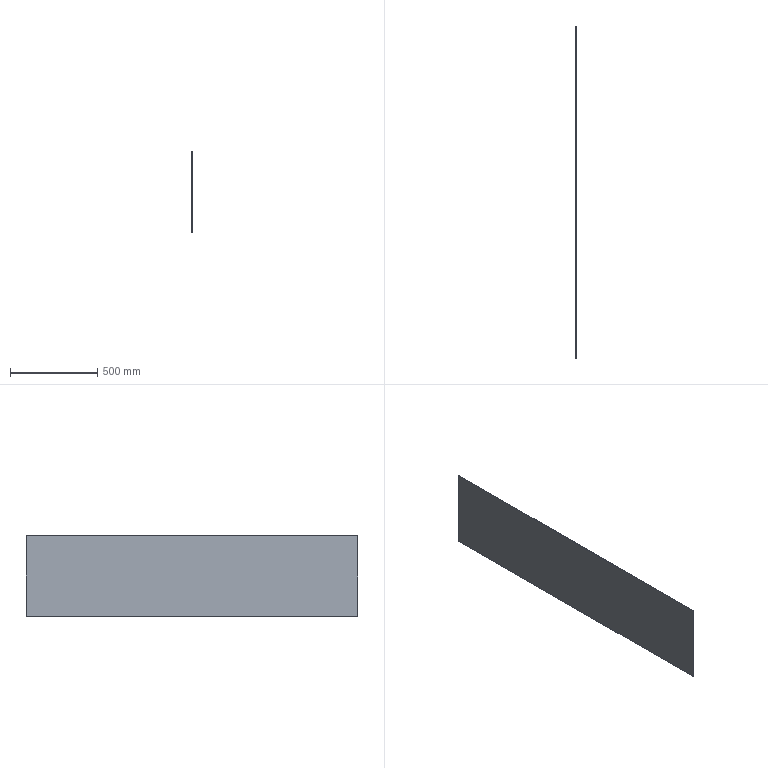Component | SolidWorks | SideBottomPlate-1 | 1 solid | 6 faces | box 2 x 1900 x 460 mm | volume 1748000 mm3 | plane 6 | material Plain Carbon Steel
STEP:
#1=CARTESIAN_POINT('',(-18.861,73.955,-5.218));
#2=VERTEX_POINT('',#1);
#3=CARTESIAN_POINT('',(-18.861,-0.848,-5.218));
#4=VERTEX_POINT('',#3);
#5=CARTESIAN_POINT('',(-18.861,73.955,-5.218));
#6=DIRECTION('',(-0.,-1.,0.));
#7=VECTOR('',#6,39.37);
#8=LINE('',#5,#7);
#9=EDGE_CURVE('',#2,#4,#8,.T.);
#10=ORIENTED_EDGE('',*,*,#9,.F.);
#11=CARTESIAN_POINT('',(-18.782,73.955,-5.218));
#12=VERTEX_POINT('',#11);
#13=CARTESIAN_POINT('',(-18.782,73.955,-5.218));
#14=DIRECTION('',(-1.,0.,-0.));
#15=VECTOR('',#14,39.37);
#16=LINE('',#13,#15);
#17=EDGE_CURVE('',#12,#2,#16,.T.);
#18=ORIENTED_EDGE('',*,*,#17,.F.);
#19=CARTESIAN_POINT('',(-18.782,-0.848,-5.218));
#20=VERTEX_POINT('',#19);
#21=CARTESIAN_POINT('',(-18.782,73.955,-5.218));
#22=DIRECTION('',(-0.,-1.,0.));
#23=VECTOR('',#22,39.37);
#24=LINE('',#21,#23);
#25=EDGE_CURVE('',#12,#20,#24,.T.);
#26=ORIENTED_EDGE('',*,*,#25,.T.);
#27=CARTESIAN_POINT('',(-18.782,-0.848,-5.218));
#28=DIRECTION('',(-1.,0.,-0.));
#29=VECTOR('',#28,39.37);
#30=LINE('',#27,#29);
#31=EDGE_CURVE('',#20,#4,#30,.T.);
#32=ORIENTED_EDGE('',*,*,#31,.T.);
#33=EDGE_LOOP('',(#10,#18,#26,#32));
#34=FACE_OUTER_BOUND('',#33,.T.);
#35=CARTESIAN_POINT('',(-18.782,73.955,-5.218));
#36=DIRECTION('',(0.,-0.,-1.));
#37=DIRECTION('',(-0.,-1.,0.));
#38=AXIS2_PLACEMENT_3D('',#35,#36,#37);
#39=PLANE('',#38);
#40=ADVANCED_FACE('',(#34),#39,.T.);
#41=CARTESIAN_POINT('',(-18.861,73.955,12.893));
#42=VERTEX_POINT('',#41);
#43=CARTESIAN_POINT('',(-18.861,73.955,-5.218));
#44=DIRECTION('',(0.,-0.,-1.));
#45=VECTOR('',#44,39.37);
#46=LINE('',#43,#45);
#47=EDGE_CURVE('',#42,#2,#46,.T.);
#48=ORIENTED_EDGE('',*,*,#47,.F.);
#49=CARTESIAN_POINT('',(-18.782,73.955,12.893));
#50=VERTEX_POINT('',#49);
#51=CARTESIAN_POINT('',(-18.782,73.955,12.893));
#52=DIRECTION('',(-1.,0.,-0.));
#53=VECTOR('',#52,39.37);
#54=LINE('',#51,#53);
#55=EDGE_CURVE('',#50,#42,#54,.T.);
#56=ORIENTED_EDGE('',*,*,#55,.F.);
#57=CARTESIAN_POINT('',(-18.782,73.955,-5.218));
#58=DIRECTION('',(0.,-0.,-1.));
#59=VECTOR('',#58,39.37);
#60=LINE('',#57,#59);
#61=EDGE_CURVE('',#50,#12,#60,.T.);
#62=ORIENTED_EDGE('',*,*,#61,.T.);
#63=ORIENTED_EDGE('',*,*,#17,.T.);
#64=EDGE_LOOP('',(#48,#56,#62,#63));
#65=FACE_OUTER_BOUND('',#64,.T.);
#66=CARTESIAN_POINT('',(-18.782,73.955,-5.218));
#67=DIRECTION('',(0.,1.,-0.));
#68=DIRECTION('',(-1.,0.,-0.));
#69=AXIS2_PLACEMENT_3D('',#66,#67,#68);
#70=PLANE('',#69);
#71=ADVANCED_FACE('',(#65),#70,.T.);
#72=CARTESIAN_POINT('',(-18.861,-0.848,12.893));
#73=VERTEX_POINT('',#72);
#74=CARTESIAN_POINT('',(-18.861,73.955,12.893));
#75=DIRECTION('',(0.,1.,-0.));
#76=VECTOR('',#75,39.37);
#77=LINE('',#74,#76);
#78=EDGE_CURVE('',#73,#42,#77,.T.);
#79=ORIENTED_EDGE('',*,*,#78,.F.);
#80=CARTESIAN_POINT('',(-18.782,-0.848,12.893));
#81=VERTEX_POINT('',#80);
#82=CARTESIAN_POINT('',(-18.782,-0.848,12.893));
#83=DIRECTION('',(-1.,0.,-0.));
#84=VECTOR('',#83,39.37);
#85=LINE('',#82,#84);
#86=EDGE_CURVE('',#81,#73,#85,.T.);
#87=ORIENTED_EDGE('',*,*,#86,.F.);
#88=CARTESIAN_POINT('',(-18.782,73.955,12.893));
#89=DIRECTION('',(0.,1.,-0.));
#90=VECTOR('',#89,39.37);
#91=LINE('',#88,#90);
#92=EDGE_CURVE('',#81,#50,#91,.T.);
#93=ORIENTED_EDGE('',*,*,#92,.T.);
#94=ORIENTED_EDGE('',*,*,#55,.T.);
#95=EDGE_LOOP('',(#79,#87,#93,#94));
#96=FACE_OUTER_BOUND('',#95,.T.);
#97=CARTESIAN_POINT('',(-18.782,73.955,12.893));
#98=DIRECTION('',(-0.,0.,1.));
#99=DIRECTION('',(0.,1.,-0.));
#100=AXIS2_PLACEMENT_3D('',#97,#98,#99);
#101=PLANE('',#100);
#102=ADVANCED_FACE('',(#96),#101,.T.);
#103=CARTESIAN_POINT('',(-18.861,-0.848,-5.218));
#104=DIRECTION('',(-0.,0.,1.));
#105=VECTOR('',#104,39.37);
#106=LINE('',#103,#105);
#107=EDGE_CURVE('',#4,#73,#106,.T.);
#108=ORIENTED_EDGE('',*,*,#107,.F.);
#109=ORIENTED_EDGE('',*,*,#31,.F.);
#110=CARTESIAN_POINT('',(-18.782,-0.848,-5.218));
#111=DIRECTION('',(-0.,0.,1.));
#112=VECTOR('',#111,39.37);
#113=LINE('',#110,#112);
#114=EDGE_CURVE('',#20,#81,#113,.T.);
#115=ORIENTED_EDGE('',*,*,#114,.T.);
#116=ORIENTED_EDGE('',*,*,#86,.T.);
#117=EDGE_LOOP('',(#108,#109,#115,#116));
#118=FACE_OUTER_BOUND('',#117,.T.);
#119=CARTESIAN_POINT('',(-18.782,-0.848,-5.218));
#120=DIRECTION('',(-0.,-1.,0.));
#121=DIRECTION('',(1.,-0.,0.));
#122=AXIS2_PLACEMENT_3D('',#119,#120,#121);
#123=PLANE('',#122);
#124=ADVANCED_FACE('',(#118),#123,.T.);
#125=ORIENTED_EDGE('',*,*,#25,.F.);
#126=ORIENTED_EDGE('',*,*,#61,.F.);
#127=ORIENTED_EDGE('',*,*,#92,.F.);
#128=ORIENTED_EDGE('',*,*,#114,.F.);
#129=EDGE_LOOP('',(#125,#126,#127,#128));
#130=FACE_OUTER_BOUND('',#129,.T.);
#131=CARTESIAN_POINT('',(-18.782,71.776,-1.6));
#132=DIRECTION('',(-1.,0.,-0.));
#133=DIRECTION('',(-0.,0.,1.));
#134=AXIS2_PLACEMENT_3D('',#131,#132,#133);
#135=PLANE('',#134);
#136=ADVANCED_FACE('',(#130),#135,.F.);
#137=ORIENTED_EDGE('',*,*,#9,.T.);
#138=ORIENTED_EDGE('',*,*,#107,.T.);
#139=ORIENTED_EDGE('',*,*,#78,.T.);
#140=ORIENTED_EDGE('',*,*,#47,.T.);
#141=EDGE_LOOP('',(#137,#138,#139,#140));
#142=FACE_OUTER_BOUND('',#141,.T.);
#143=CARTESIAN_POINT('',(-18.861,71.776,-1.6));
#144=DIRECTION('',(-1.,0.,-0.));
#145=DIRECTION('',(-0.,0.,1.));
#146=AXIS2_PLACEMENT_3D('',#143,#144,#145);
#147=PLANE('',#146);
#148=ADVANCED_FACE('',(#142),#147,.T.);
#149=CLOSED_SHELL('',(#40,#71,#102,#124,#136,#148));
#150=MANIFOLD_SOLID_BREP('',#149);
#151=CARTESIAN_POINT('',(0.,0.,0.));
#152=DIRECTION('',(0.,0.,1.));
#153=DIRECTION('',(1.,0.,0.));
#154=AXIS2_PLACEMENT_3D('',#151,#152,#153);
#155=(LENGTH_UNIT()NAMED_UNIT(*)SI_UNIT($,.METRE.));
#156=LENGTH_MEASURE_WITH_UNIT(LENGTH_MEASURE(0.0254),#155);
#157=DIMENSIONAL_EXPONENTS(1.,0.,0.,0.,0.,0.,0.);
#158=(CONVERSION_BASED_UNIT('',#156)LENGTH_UNIT()NAMED_UNIT(#157));
#159=UNCERTAINTY_MEASURE_WITH_UNIT(LENGTH_MEASURE(0.00001),#158,'','');
#160=(NAMED_UNIT(*)PLANE_ANGLE_UNIT()SI_UNIT($,.RADIAN.));
#161=(NAMED_UNIT(*)SI_UNIT($,.STERADIAN.)SOLID_ANGLE_UNIT());
#162=(GEOMETRIC_REPRESENTATION_CONTEXT(3)GLOBAL_UNCERTAINTY_ASSIGNED_CONTEXT((#159))GLOBAL_UNIT_ASSIGNED_CONTEXT((#158,#160,#161))REPRESENTATION_CONTEXT('',''));
#163=ADVANCED_BREP_SHAPE_REPRESENTATION('',(#150,#154),#162);
#164=COLOUR_RGB('',0.7922,0.8196,0.9333);
#165=FILL_AREA_STYLE_COLOUR('',#164);
#166=FILL_AREA_STYLE('',(#165));
#167=SURFACE_STYLE_FILL_AREA(#166);
#168=SURFACE_SIDE_STYLE('',(#167));
#169=SURFACE_STYLE_USAGE(.BOTH.,#168);
#170=PRESENTATION_STYLE_ASSIGNMENT((#169));
#171=STYLED_ITEM('',(#170),#150);
#172=PRESENTATION_LAYER_ASSIGNMENT('','',(#171));
#173=(LENGTH_UNIT()NAMED_UNIT(*)SI_UNIT($,.METRE.));
#174=LENGTH_MEASURE_WITH_UNIT(LENGTH_MEASURE(0.0254),#173);
#175=DIMENSIONAL_EXPONENTS(1.,0.,0.,0.,0.,0.,0.);
#176=(CONVERSION_BASED_UNIT('',#174)LENGTH_UNIT()NAMED_UNIT(#175));
#177=UNCERTAINTY_MEASURE_WITH_UNIT(LENGTH_MEASURE(0.00001),#176,'','');
#178=(NAMED_UNIT(*)PLANE_ANGLE_UNIT()SI_UNIT($,.RADIAN.));
#179=(NAMED_UNIT(*)SI_UNIT($,.STERADIAN.)SOLID_ANGLE_UNIT());
#180=(GEOMETRIC_REPRESENTATION_CONTEXT(3)GLOBAL_UNCERTAINTY_ASSIGNED_CONTEXT((#177))GLOBAL_UNIT_ASSIGNED_CONTEXT((#176,#178,#179))REPRESENTATION_CONTEXT('',''));
#181=MECHANICAL_DESIGN_GEOMETRIC_PRESENTATION_REPRESENTATION('',(#171),#180);